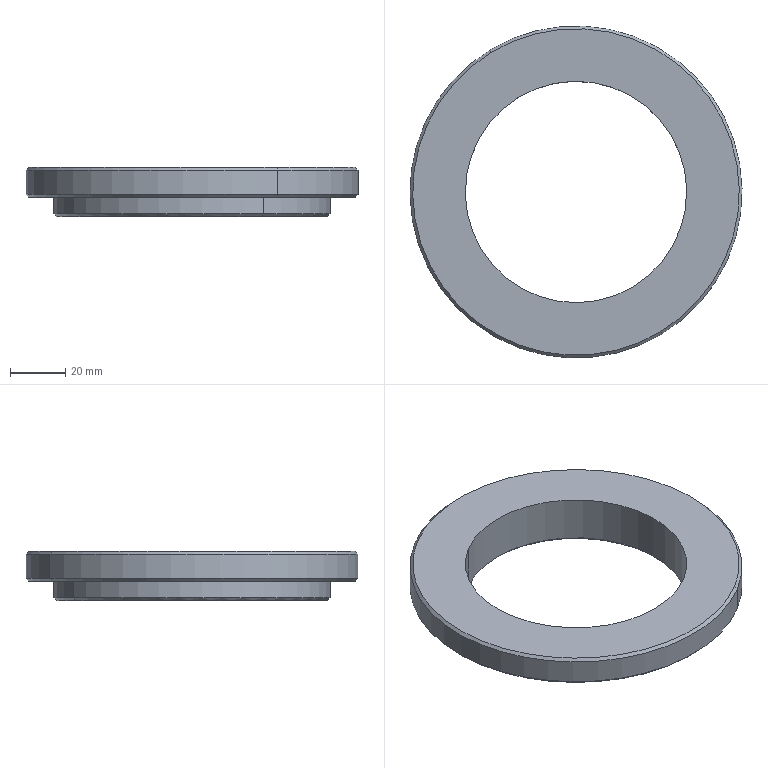Component | SolidWorks | PartAssemblyInLowerHousing-1_LowSpeedAxisAssembly-1_SleeveOnLowSpeedAxis-1 | 1 solid | 17 faces | box 120 x 120 x 17.75 mm | volume 86679 mm3 | cone 8 | cylinder 6 | plane 3 | commonest cylinder face diameters 100 x2 80 x2 120 x2
build123d program:
from build123d import *

# Parameters (mm, degrees)
CHAMFER1_SIZE = 1


with BuildPart() as part:
    # Sketch1 → Revolve1 (revolve)
    with BuildSketch(Plane.XY, mode=Mode.PRIVATE) as revolve1_sk:
        Polygon((0, 60), (0, 40), (17.75, 40), (17.75, 50), (10.75, 50), (10.75, 60), align=None)
    revolve(revolve1_sk.sketch.rotate(Axis((0, 0, 0), (1, 0, 0)), 90), axis=Axis((0, 0, 0), (1, 0, 0)))

    # Chamfer1
    chamfer1_edges = [part.edges().sort_by_distance(p)[0] for p in [
        (10.75, 0, -60),
        (17.75, 0, -50),
        (17.75, 0, -40),
        (0, 0, -60),
    ]]
    chamfer(chamfer1_edges, length=CHAMFER1_SIZE)


solid = part.part

# Placed as in the assembly
solid = solid.moved(Location((1140.83, 1268.591, 1539.214), (0, 90, 0)))
STEP:
#1=CARTESIAN_POINT('',(43.714,51.933,60.599));
#2=VERTEX_POINT('',#1);
#3=CARTESIAN_POINT('',(46.116,47.956,60.599));
#4=VERTEX_POINT('',#3);
#5=CARTESIAN_POINT('',(44.915,49.945,60.599));
#6=DIRECTION('',(-0.,0.,1.));
#7=DIRECTION('',(0.517,-0.856,0.));
#8=AXIS2_PLACEMENT_3D('',#5,#6,#7);
#9=CIRCLE('',#8,2.323);
#10=EDGE_CURVE('',#2,#4,#9,.T.);
#11=ORIENTED_EDGE('',*,*,#10,.F.);
#12=CARTESIAN_POINT('',(43.693,51.966,60.56));
#13=VERTEX_POINT('',#12);
#14=CARTESIAN_POINT('',(43.714,51.933,60.599));
#15=DIRECTION('',(-0.3656,0.6053,-0.7071));
#16=VECTOR('',#15,39.37);
#17=LINE('',#14,#16);
#18=EDGE_CURVE('',#2,#13,#17,.T.);
#19=ORIENTED_EDGE('',*,*,#18,.T.);
#20=CARTESIAN_POINT('',(46.136,47.923,60.56));
#21=VERTEX_POINT('',#20);
#22=CARTESIAN_POINT('',(44.915,49.945,60.56));
#23=DIRECTION('',(0.,-0.,-1.));
#24=DIRECTION('',(0.517,-0.856,0.));
#25=AXIS2_PLACEMENT_3D('',#22,#23,#24);
#26=CIRCLE('',#25,2.362);
#27=EDGE_CURVE('',#21,#13,#26,.T.);
#28=ORIENTED_EDGE('',*,*,#27,.F.);
#29=CARTESIAN_POINT('',(46.116,47.956,60.599));
#30=DIRECTION('',(0.3656,-0.6053,-0.7071));
#31=VECTOR('',#30,39.37);
#32=LINE('',#29,#31);
#33=EDGE_CURVE('',#4,#21,#32,.T.);
#34=ORIENTED_EDGE('',*,*,#33,.F.);
#35=EDGE_LOOP('',(#11,#19,#28,#34));
#36=FACE_OUTER_BOUND('',#35,.T.);
#37=CARTESIAN_POINT('',(44.915,49.945,60.599));
#38=DIRECTION('',(0.,-0.,-1.));
#39=DIRECTION('',(0.517,-0.856,0.));
#40=AXIS2_PLACEMENT_3D('',#37,#38,#39);
#41=CONICAL_SURFACE('',#40,2.323,0.7854);
#42=ADVANCED_FACE('',(#36),#41,.T.);
#43=CARTESIAN_POINT('',(46.116,47.956,60.176));
#44=VERTEX_POINT('',#43);
#45=CARTESIAN_POINT('',(43.714,51.933,60.176));
#46=VERTEX_POINT('',#45);
#47=CARTESIAN_POINT('',(44.915,49.945,60.176));
#48=DIRECTION('',(0.,-0.,-1.));
#49=DIRECTION('',(-0.517,0.856,0.));
#50=AXIS2_PLACEMENT_3D('',#47,#48,#49);
#51=CIRCLE('',#50,2.323);
#52=EDGE_CURVE('',#44,#46,#51,.T.);
#53=ORIENTED_EDGE('',*,*,#52,.F.);
#54=CARTESIAN_POINT('',(46.136,47.923,60.215));
#55=VERTEX_POINT('',#54);
#56=CARTESIAN_POINT('',(46.136,47.923,60.215));
#57=DIRECTION('',(0.3656,-0.6053,0.7071));
#58=VECTOR('',#57,39.37);
#59=LINE('',#56,#58);
#60=EDGE_CURVE('',#44,#55,#59,.T.);
#61=ORIENTED_EDGE('',*,*,#60,.T.);
#62=CARTESIAN_POINT('',(43.693,51.966,60.215));
#63=VERTEX_POINT('',#62);
#64=CARTESIAN_POINT('',(44.915,49.945,60.215));
#65=DIRECTION('',(-0.,0.,1.));
#66=DIRECTION('',(-0.517,0.856,0.));
#67=AXIS2_PLACEMENT_3D('',#64,#65,#66);
#68=CIRCLE('',#67,2.362);
#69=EDGE_CURVE('',#63,#55,#68,.T.);
#70=ORIENTED_EDGE('',*,*,#69,.F.);
#71=CARTESIAN_POINT('',(43.693,51.966,60.215));
#72=DIRECTION('',(-0.3656,0.6053,0.7071));
#73=VECTOR('',#72,39.37);
#74=LINE('',#71,#73);
#75=EDGE_CURVE('',#46,#63,#74,.T.);
#76=ORIENTED_EDGE('',*,*,#75,.F.);
#77=EDGE_LOOP('',(#53,#61,#70,#76));
#78=FACE_OUTER_BOUND('',#77,.T.);
#79=CARTESIAN_POINT('',(44.915,49.945,60.215));
#80=DIRECTION('',(-0.,0.,1.));
#81=DIRECTION('',(-0.517,0.856,0.));
#82=AXIS2_PLACEMENT_3D('',#79,#80,#81);
#83=CONICAL_SURFACE('',#82,2.362,0.7854);
#84=ADVANCED_FACE('',(#78),#83,.T.);
#85=CARTESIAN_POINT('',(45.912,48.293,59.9));
#86=VERTEX_POINT('',#85);
#87=CARTESIAN_POINT('',(43.917,51.596,59.9));
#88=VERTEX_POINT('',#87);
#89=CARTESIAN_POINT('',(44.915,49.945,59.9));
#90=DIRECTION('',(0.,-0.,-1.));
#91=DIRECTION('',(-0.517,0.856,0.));
#92=AXIS2_PLACEMENT_3D('',#89,#90,#91);
#93=CIRCLE('',#92,1.929);
#94=EDGE_CURVE('',#86,#88,#93,.T.);
#95=ORIENTED_EDGE('',*,*,#94,.F.);
#96=CARTESIAN_POINT('',(45.932,48.26,59.94));
#97=VERTEX_POINT('',#96);
#98=CARTESIAN_POINT('',(45.932,48.26,59.94));
#99=DIRECTION('',(0.3656,-0.6053,0.7071));
#100=VECTOR('',#99,39.37);
#101=LINE('',#98,#100);
#102=EDGE_CURVE('',#86,#97,#101,.T.);
#103=ORIENTED_EDGE('',*,*,#102,.T.);
#104=CARTESIAN_POINT('',(43.897,51.629,59.94));
#105=VERTEX_POINT('',#104);
#106=CARTESIAN_POINT('',(44.915,49.945,59.94));
#107=DIRECTION('',(-0.,0.,1.));
#108=DIRECTION('',(-0.517,0.856,0.));
#109=AXIS2_PLACEMENT_3D('',#106,#107,#108);
#110=CIRCLE('',#109,1.969);
#111=EDGE_CURVE('',#105,#97,#110,.T.);
#112=ORIENTED_EDGE('',*,*,#111,.F.);
#113=CARTESIAN_POINT('',(43.897,51.629,59.94));
#114=DIRECTION('',(-0.3656,0.6053,0.7071));
#115=VECTOR('',#114,39.37);
#116=LINE('',#113,#115);
#117=EDGE_CURVE('',#88,#105,#116,.T.);
#118=ORIENTED_EDGE('',*,*,#117,.F.);
#119=EDGE_LOOP('',(#95,#103,#112,#118));
#120=FACE_OUTER_BOUND('',#119,.T.);
#121=CARTESIAN_POINT('',(44.915,49.945,59.94));
#122=DIRECTION('',(-0.,0.,1.));
#123=DIRECTION('',(-0.517,0.856,0.));
#124=AXIS2_PLACEMENT_3D('',#121,#122,#123);
#125=CONICAL_SURFACE('',#124,1.969,0.7854);
#126=ADVANCED_FACE('',(#120),#125,.T.);
#127=CARTESIAN_POINT('',(44.1,51.292,59.94));
#128=VERTEX_POINT('',#127);
#129=CARTESIAN_POINT('',(45.729,48.597,59.94));
#130=VERTEX_POINT('',#129);
#131=CARTESIAN_POINT('',(44.915,49.945,59.94));
#132=DIRECTION('',(0.,-0.,-1.));
#133=DIRECTION('',(-0.517,0.856,0.));
#134=AXIS2_PLACEMENT_3D('',#131,#132,#133);
#135=CIRCLE('',#134,1.575);
#136=EDGE_CURVE('',#128,#130,#135,.T.);
#137=ORIENTED_EDGE('',*,*,#136,.F.);
#138=CARTESIAN_POINT('',(44.08,51.326,59.9));
#139=VERTEX_POINT('',#138);
#140=CARTESIAN_POINT('',(44.08,51.326,59.9));
#141=DIRECTION('',(-0.3656,0.6053,-0.7071));
#142=VECTOR('',#141,39.37);
#143=LINE('',#140,#142);
#144=EDGE_CURVE('',#128,#139,#143,.T.);
#145=ORIENTED_EDGE('',*,*,#144,.T.);
#146=CARTESIAN_POINT('',(45.749,48.563,59.9));
#147=VERTEX_POINT('',#146);
#148=CARTESIAN_POINT('',(44.915,49.945,59.9));
#149=DIRECTION('',(-0.,0.,1.));
#150=DIRECTION('',(-0.517,0.856,0.));
#151=AXIS2_PLACEMENT_3D('',#148,#149,#150);
#152=CIRCLE('',#151,1.614);
#153=EDGE_CURVE('',#147,#139,#152,.T.);
#154=ORIENTED_EDGE('',*,*,#153,.F.);
#155=CARTESIAN_POINT('',(45.749,48.563,59.9));
#156=DIRECTION('',(0.3656,-0.6053,-0.7071));
#157=VECTOR('',#156,39.37);
#158=LINE('',#155,#157);
#159=EDGE_CURVE('',#130,#147,#158,.T.);
#160=ORIENTED_EDGE('',*,*,#159,.F.);
#161=EDGE_LOOP('',(#137,#145,#154,#160));
#162=FACE_OUTER_BOUND('',#161,.T.);
#163=CARTESIAN_POINT('',(44.915,49.945,59.9));
#164=DIRECTION('',(0.,-0.,-1.));
#165=DIRECTION('',(0.517,-0.856,0.));
#166=AXIS2_PLACEMENT_3D('',#163,#164,#165);
#167=CONICAL_SURFACE('',#166,1.614,0.7854);
#168=ADVANCED_FACE('',(#162),#167,.F.);
#169=ORIENTED_EDGE('',*,*,#111,.T.);
#170=CARTESIAN_POINT('',(45.932,48.26,60.176));
#171=VERTEX_POINT('',#170);
#172=CARTESIAN_POINT('',(45.932,48.26,60.599));
#173=DIRECTION('',(-0.,0.,1.));
#174=VECTOR('',#173,39.37);
#175=LINE('',#172,#174);
#176=EDGE_CURVE('',#97,#171,#175,.T.);
#177=ORIENTED_EDGE('',*,*,#176,.T.);
#178=CARTESIAN_POINT('',(43.897,51.629,60.176));
#179=VERTEX_POINT('',#178);
#180=CARTESIAN_POINT('',(44.915,49.945,60.176));
#181=DIRECTION('',(-0.,0.,1.));
#182=DIRECTION('',(-0.517,0.856,0.));
#183=AXIS2_PLACEMENT_3D('',#180,#181,#182);
#184=CIRCLE('',#183,1.969);
#185=EDGE_CURVE('',#179,#171,#184,.T.);
#186=ORIENTED_EDGE('',*,*,#185,.F.);
#187=CARTESIAN_POINT('',(43.897,51.629,60.599));
#188=DIRECTION('',(-0.,0.,1.));
#189=VECTOR('',#188,39.37);
#190=LINE('',#187,#189);
#191=EDGE_CURVE('',#105,#179,#190,.T.);
#192=ORIENTED_EDGE('',*,*,#191,.F.);
#193=EDGE_LOOP('',(#169,#177,#186,#192));
#194=FACE_OUTER_BOUND('',#193,.T.);
#195=CARTESIAN_POINT('',(44.915,49.945,60.599));
#196=DIRECTION('',(-0.,0.,1.));
#197=DIRECTION('',(-0.517,0.856,0.));
#198=AXIS2_PLACEMENT_3D('',#195,#196,#197);
#199=CYLINDRICAL_SURFACE('',#198,1.969);
#200=ADVANCED_FACE('',(#194),#199,.T.);
#201=ORIENTED_EDGE('',*,*,#136,.T.);
#202=CARTESIAN_POINT('',(45.729,48.597,60.599));
#203=VERTEX_POINT('',#202);
#204=CARTESIAN_POINT('',(45.729,48.597,60.599));
#205=DIRECTION('',(-0.,0.,1.));
#206=VECTOR('',#205,39.37);
#207=LINE('',#204,#206);
#208=EDGE_CURVE('',#130,#203,#207,.T.);
#209=ORIENTED_EDGE('',*,*,#208,.T.);
#210=CARTESIAN_POINT('',(44.1,51.292,60.599));
#211=VERTEX_POINT('',#210);
#212=CARTESIAN_POINT('',(44.915,49.945,60.599));
#213=DIRECTION('',(-0.,0.,1.));
#214=DIRECTION('',(-0.517,0.856,0.));
#215=AXIS2_PLACEMENT_3D('',#212,#213,#214);
#216=CIRCLE('',#215,1.575);
#217=EDGE_CURVE('',#203,#211,#216,.T.);
#218=ORIENTED_EDGE('',*,*,#217,.T.);
#219=CARTESIAN_POINT('',(44.1,51.292,60.599));
#220=DIRECTION('',(-0.,0.,1.));
#221=VECTOR('',#220,39.37);
#222=LINE('',#219,#221);
#223=EDGE_CURVE('',#128,#211,#222,.T.);
#224=ORIENTED_EDGE('',*,*,#223,.F.);
#225=EDGE_LOOP('',(#201,#209,#218,#224));
#226=FACE_OUTER_BOUND('',#225,.T.);
#227=CARTESIAN_POINT('',(44.915,49.945,60.599));
#228=DIRECTION('',(-0.,0.,1.));
#229=DIRECTION('',(-0.517,0.856,0.));
#230=AXIS2_PLACEMENT_3D('',#227,#228,#229);
#231=CYLINDRICAL_SURFACE('',#230,1.575);
#232=ADVANCED_FACE('',(#226),#231,.F.);
#233=ORIENTED_EDGE('',*,*,#69,.T.);
#234=CARTESIAN_POINT('',(46.136,47.923,60.599));
#235=DIRECTION('',(-0.,0.,1.));
#236=VECTOR('',#235,39.37);
#237=LINE('',#234,#236);
#238=EDGE_CURVE('',#55,#21,#237,.T.);
#239=ORIENTED_EDGE('',*,*,#238,.T.);
#240=ORIENTED_EDGE('',*,*,#27,.T.);
#241=CARTESIAN_POINT('',(43.693,51.966,60.599));
#242=DIRECTION('',(-0.,0.,1.));
#243=VECTOR('',#242,39.37);
#244=LINE('',#241,#243);
#245=EDGE_CURVE('',#63,#13,#244,.T.);
#246=ORIENTED_EDGE('',*,*,#245,.F.);
#247=EDGE_LOOP('',(#233,#239,#240,#246));
#248=FACE_OUTER_BOUND('',#247,.T.);
#249=CARTESIAN_POINT('',(44.915,49.945,60.599));
#250=DIRECTION('',(-0.,0.,1.));
#251=DIRECTION('',(-0.517,0.856,0.));
#252=AXIS2_PLACEMENT_3D('',#249,#250,#251);
#253=CYLINDRICAL_SURFACE('',#252,2.362);
#254=ADVANCED_FACE('',(#248),#253,.T.);
#255=ORIENTED_EDGE('',*,*,#238,.F.);
#256=CARTESIAN_POINT('',(44.915,49.945,60.215));
#257=DIRECTION('',(-0.,0.,1.));
#258=DIRECTION('',(-0.517,0.856,0.));
#259=AXIS2_PLACEMENT_3D('',#256,#257,#258);
#260=CIRCLE('',#259,2.362);
#261=EDGE_CURVE('',#55,#63,#260,.T.);
#262=ORIENTED_EDGE('',*,*,#261,.T.);
#263=ORIENTED_EDGE('',*,*,#245,.T.);
#264=CARTESIAN_POINT('',(44.915,49.945,60.56));
#265=DIRECTION('',(0.,-0.,-1.));
#266=DIRECTION('',(0.517,-0.856,0.));
#267=AXIS2_PLACEMENT_3D('',#264,#265,#266);
#268=CIRCLE('',#267,2.362);
#269=EDGE_CURVE('',#13,#21,#268,.T.);
#270=ORIENTED_EDGE('',*,*,#269,.T.);
#271=EDGE_LOOP('',(#255,#262,#263,#270));
#272=FACE_OUTER_BOUND('',#271,.T.);
#273=CARTESIAN_POINT('',(44.915,49.945,60.599));
#274=DIRECTION('',(-0.,0.,1.));
#275=DIRECTION('',(-0.517,0.856,0.));
#276=AXIS2_PLACEMENT_3D('',#273,#274,#275);
#277=CYLINDRICAL_SURFACE('',#276,2.362);
#278=ADVANCED_FACE('',(#272),#277,.T.);
#279=CARTESIAN_POINT('',(44.915,49.945,60.599));
#280=DIRECTION('',(-0.,0.,1.));
#281=DIRECTION('',(0.517,-0.856,0.));
#282=AXIS2_PLACEMENT_3D('',#279,#280,#281);
#283=CIRCLE('',#282,2.323);
#284=EDGE_CURVE('',#4,#2,#283,.T.);
#285=ORIENTED_EDGE('',*,*,#284,.T.);
#286=ORIENTED_EDGE('',*,*,#10,.T.);
#287=EDGE_LOOP('',(#285,#286));
#288=FACE_OUTER_BOUND('',#287,.T.);
#289=CARTESIAN_POINT('',(44.915,49.945,60.599));
#290=DIRECTION('',(-0.,0.,1.));
#291=DIRECTION('',(-0.517,0.856,0.));
#292=AXIS2_PLACEMENT_3D('',#289,#290,#291);
#293=CIRCLE('',#292,1.575);
#294=EDGE_CURVE('',#211,#203,#293,.T.);
#295=ORIENTED_EDGE('',*,*,#294,.F.);
#296=ORIENTED_EDGE('',*,*,#217,.F.);
#297=EDGE_LOOP('',(#295,#296));
#298=FACE_BOUND('',#297,.T.);
#299=CARTESIAN_POINT('',(42.893,48.723,60.599));
#300=DIRECTION('',(0.,-0.,-1.));
#301=DIRECTION('',(0.517,-0.856,0.));
#302=AXIS2_PLACEMENT_3D('',#299,#300,#301);
#303=PLANE('',#302);
#304=ADVANCED_FACE('',(#288,#298),#303,.F.);
#305=ORIENTED_EDGE('',*,*,#208,.F.);
#306=CARTESIAN_POINT('',(44.915,49.945,59.94));
#307=DIRECTION('',(0.,-0.,-1.));
#308=DIRECTION('',(-0.517,0.856,0.));
#309=AXIS2_PLACEMENT_3D('',#306,#307,#308);
#310=CIRCLE('',#309,1.575);
#311=EDGE_CURVE('',#130,#128,#310,.T.);
#312=ORIENTED_EDGE('',*,*,#311,.T.);
#313=ORIENTED_EDGE('',*,*,#223,.T.);
#314=ORIENTED_EDGE('',*,*,#294,.T.);
#315=EDGE_LOOP('',(#305,#312,#313,#314));
#316=FACE_OUTER_BOUND('',#315,.T.);
#317=CARTESIAN_POINT('',(44.915,49.945,60.599));
#318=DIRECTION('',(-0.,0.,1.));
#319=DIRECTION('',(-0.517,0.856,0.));
#320=AXIS2_PLACEMENT_3D('',#317,#318,#319);
#321=CYLINDRICAL_SURFACE('',#320,1.575);
#322=ADVANCED_FACE('',(#316),#321,.F.);
#323=ORIENTED_EDGE('',*,*,#153,.T.);
#324=CARTESIAN_POINT('',(44.915,49.945,59.9));
#325=DIRECTION('',(-0.,0.,1.));
#326=DIRECTION('',(-0.517,0.856,0.));
#327=AXIS2_PLACEMENT_3D('',#324,#325,#326);
#328=CIRCLE('',#327,1.614);
#329=EDGE_CURVE('',#139,#147,#328,.T.);
#330=ORIENTED_EDGE('',*,*,#329,.T.);
#331=EDGE_LOOP('',(#323,#330));
#332=FACE_BOUND('',#331,.T.);
#333=CARTESIAN_POINT('',(44.915,49.945,59.9));
#334=DIRECTION('',(0.,-0.,-1.));
#335=DIRECTION('',(-0.517,0.856,0.));
#336=AXIS2_PLACEMENT_3D('',#333,#334,#335);
#337=CIRCLE('',#336,1.929);
#338=EDGE_CURVE('',#88,#86,#337,.T.);
#339=ORIENTED_EDGE('',*,*,#338,.T.);
#340=ORIENTED_EDGE('',*,*,#94,.T.);
#341=EDGE_LOOP('',(#339,#340));
#342=FACE_OUTER_BOUND('',#341,.T.);
#343=CARTESIAN_POINT('',(43.567,49.13,59.9));
#344=DIRECTION('',(-0.,0.,1.));
#345=DIRECTION('',(-0.517,0.856,-0.));
#346=AXIS2_PLACEMENT_3D('',#343,#344,#345);
#347=PLANE('',#346);
#348=ADVANCED_FACE('',(#332,#342),#347,.F.);
#349=ORIENTED_EDGE('',*,*,#176,.F.);
#350=CARTESIAN_POINT('',(44.915,49.945,59.94));
#351=DIRECTION('',(-0.,0.,1.));
#352=DIRECTION('',(-0.517,0.856,0.));
#353=AXIS2_PLACEMENT_3D('',#350,#351,#352);
#354=CIRCLE('',#353,1.969);
#355=EDGE_CURVE('',#97,#105,#354,.T.);
#356=ORIENTED_EDGE('',*,*,#355,.T.);
#357=ORIENTED_EDGE('',*,*,#191,.T.);
#358=CARTESIAN_POINT('',(44.915,49.945,60.176));
#359=DIRECTION('',(-0.,0.,1.));
#360=DIRECTION('',(-0.517,0.856,0.));
#361=AXIS2_PLACEMENT_3D('',#358,#359,#360);
#362=CIRCLE('',#361,1.969);
#363=EDGE_CURVE('',#171,#179,#362,.T.);
#364=ORIENTED_EDGE('',*,*,#363,.F.);
#365=EDGE_LOOP('',(#349,#356,#357,#364));
#366=FACE_OUTER_BOUND('',#365,.T.);
#367=CARTESIAN_POINT('',(44.915,49.945,60.599));
#368=DIRECTION('',(-0.,0.,1.));
#369=DIRECTION('',(-0.517,0.856,0.));
#370=AXIS2_PLACEMENT_3D('',#367,#368,#369);
#371=CYLINDRICAL_SURFACE('',#370,1.969);
#372=ADVANCED_FACE('',(#366),#371,.T.);
#373=CARTESIAN_POINT('',(44.915,49.945,60.176));
#374=DIRECTION('',(0.,-0.,-1.));
#375=DIRECTION('',(-0.517,0.856,0.));
#376=AXIS2_PLACEMENT_3D('',#373,#374,#375);
#377=CIRCLE('',#376,2.323);
#378=EDGE_CURVE('',#46,#44,#377,.T.);
#379=ORIENTED_EDGE('',*,*,#378,.T.);
#380=ORIENTED_EDGE('',*,*,#52,.T.);
#381=EDGE_LOOP('',(#379,#380));
#382=FACE_OUTER_BOUND('',#381,.T.);
#383=ORIENTED_EDGE('',*,*,#185,.T.);
#384=ORIENTED_EDGE('',*,*,#363,.T.);
#385=EDGE_LOOP('',(#383,#384));
#386=FACE_BOUND('',#385,.T.);
#387=CARTESIAN_POINT('',(43.23,48.927,60.176));
#388=DIRECTION('',(-0.,0.,1.));
#389=DIRECTION('',(-0.517,0.856,-0.));
#390=AXIS2_PLACEMENT_3D('',#387,#388,#389);
#391=PLANE('',#390);
#392=ADVANCED_FACE('',(#382,#386),#391,.F.);
#393=ORIENTED_EDGE('',*,*,#144,.F.);
#394=ORIENTED_EDGE('',*,*,#311,.F.);
#395=ORIENTED_EDGE('',*,*,#159,.T.);
#396=ORIENTED_EDGE('',*,*,#329,.F.);
#397=EDGE_LOOP('',(#393,#394,#395,#396));
#398=FACE_OUTER_BOUND('',#397,.T.);
#399=CARTESIAN_POINT('',(44.915,49.945,59.9));
#400=DIRECTION('',(0.,-0.,-1.));
#401=DIRECTION('',(0.517,-0.856,0.));
#402=AXIS2_PLACEMENT_3D('',#399,#400,#401);
#403=CONICAL_SURFACE('',#402,1.614,0.7854);
#404=ADVANCED_FACE('',(#398),#403,.F.);
#405=ORIENTED_EDGE('',*,*,#102,.F.);
#406=ORIENTED_EDGE('',*,*,#338,.F.);
#407=ORIENTED_EDGE('',*,*,#117,.T.);
#408=ORIENTED_EDGE('',*,*,#355,.F.);
#409=EDGE_LOOP('',(#405,#406,#407,#408));
#410=FACE_OUTER_BOUND('',#409,.T.);
#411=CARTESIAN_POINT('',(44.915,49.945,59.94));
#412=DIRECTION('',(-0.,0.,1.));
#413=DIRECTION('',(-0.517,0.856,0.));
#414=AXIS2_PLACEMENT_3D('',#411,#412,#413);
#415=CONICAL_SURFACE('',#414,1.969,0.7854);
#416=ADVANCED_FACE('',(#410),#415,.T.);
#417=ORIENTED_EDGE('',*,*,#60,.F.);
#418=ORIENTED_EDGE('',*,*,#378,.F.);
#419=ORIENTED_EDGE('',*,*,#75,.T.);
#420=ORIENTED_EDGE('',*,*,#261,.F.);
#421=EDGE_LOOP('',(#417,#418,#419,#420));
#422=FACE_OUTER_BOUND('',#421,.T.);
#423=CARTESIAN_POINT('',(44.915,49.945,60.215));
#424=DIRECTION('',(-0.,0.,1.));
#425=DIRECTION('',(-0.517,0.856,0.));
#426=AXIS2_PLACEMENT_3D('',#423,#424,#425);
#427=CONICAL_SURFACE('',#426,2.362,0.7854);
#428=ADVANCED_FACE('',(#422),#427,.T.);
#429=ORIENTED_EDGE('',*,*,#18,.F.);
#430=ORIENTED_EDGE('',*,*,#284,.F.);
#431=ORIENTED_EDGE('',*,*,#33,.T.);
#432=ORIENTED_EDGE('',*,*,#269,.F.);
#433=EDGE_LOOP('',(#429,#430,#431,#432));
#434=FACE_OUTER_BOUND('',#433,.T.);
#435=CARTESIAN_POINT('',(44.915,49.945,60.599));
#436=DIRECTION('',(0.,-0.,-1.));
#437=DIRECTION('',(0.517,-0.856,0.));
#438=AXIS2_PLACEMENT_3D('',#435,#436,#437);
#439=CONICAL_SURFACE('',#438,2.323,0.7854);
#440=ADVANCED_FACE('',(#434),#439,.T.);
#441=CLOSED_SHELL('',(#42,#84,#126,#168,#200,#232,#254,#278,#304,#322,#348,#372,#392,#404,#416,#428,#440));
#442=MANIFOLD_SOLID_BREP('',#441);
#443=CARTESIAN_POINT('',(0.,0.,0.));
#444=DIRECTION('',(0.,0.,1.));
#445=DIRECTION('',(1.,0.,0.));
#446=AXIS2_PLACEMENT_3D('',#443,#444,#445);
#447=(LENGTH_UNIT()NAMED_UNIT(*)SI_UNIT($,.METRE.));
#448=LENGTH_MEASURE_WITH_UNIT(LENGTH_MEASURE(0.0254),#447);
#449=DIMENSIONAL_EXPONENTS(1.,0.,0.,0.,0.,0.,0.);
#450=(CONVERSION_BASED_UNIT('',#448)LENGTH_UNIT()NAMED_UNIT(#449));
#451=UNCERTAINTY_MEASURE_WITH_UNIT(LENGTH_MEASURE(0.00001),#450,'','');
#452=(NAMED_UNIT(*)PLANE_ANGLE_UNIT()SI_UNIT($,.RADIAN.));
#453=(NAMED_UNIT(*)SI_UNIT($,.STERADIAN.)SOLID_ANGLE_UNIT());
#454=(GEOMETRIC_REPRESENTATION_CONTEXT(3)GLOBAL_UNCERTAINTY_ASSIGNED_CONTEXT((#451))GLOBAL_UNIT_ASSIGNED_CONTEXT((#450,#452,#453))REPRESENTATION_CONTEXT('',''));
#455=ADVANCED_BREP_SHAPE_REPRESENTATION('',(#442,#446),#454);
#456=COLOUR_RGB('',0.7922,0.8196,0.9333);
#457=FILL_AREA_STYLE_COLOUR('',#456);
#458=FILL_AREA_STYLE('',(#457));
#459=SURFACE_STYLE_FILL_AREA(#458);
#460=SURFACE_SIDE_STYLE('',(#459));
#461=SURFACE_STYLE_USAGE(.BOTH.,#460);
#462=PRESENTATION_STYLE_ASSIGNMENT((#461));
#463=STYLED_ITEM('',(#462),#442);
#464=(LENGTH_UNIT()NAMED_UNIT(*)SI_UNIT($,.METRE.));
#465=LENGTH_MEASURE_WITH_UNIT(LENGTH_MEASURE(0.0254),#464);
#466=DIMENSIONAL_EXPONENTS(1.,0.,0.,0.,0.,0.,0.);
#467=(CONVERSION_BASED_UNIT('',#465)LENGTH_UNIT()NAMED_UNIT(#466));
#468=UNCERTAINTY_MEASURE_WITH_UNIT(LENGTH_MEASURE(0.00001),#467,'','');
#469=(NAMED_UNIT(*)PLANE_ANGLE_UNIT()SI_UNIT($,.RADIAN.));
#470=(NAMED_UNIT(*)SI_UNIT($,.STERADIAN.)SOLID_ANGLE_UNIT());
#471=(GEOMETRIC_REPRESENTATION_CONTEXT(3)GLOBAL_UNCERTAINTY_ASSIGNED_CONTEXT((#468))GLOBAL_UNIT_ASSIGNED_CONTEXT((#467,#469,#470))REPRESENTATION_CONTEXT('',''));
#472=MECHANICAL_DESIGN_GEOMETRIC_PRESENTATION_REPRESENTATION('',(#463),#471);
#473=PRESENTATION_LAYER_ASSIGNMENT('','',(#463));